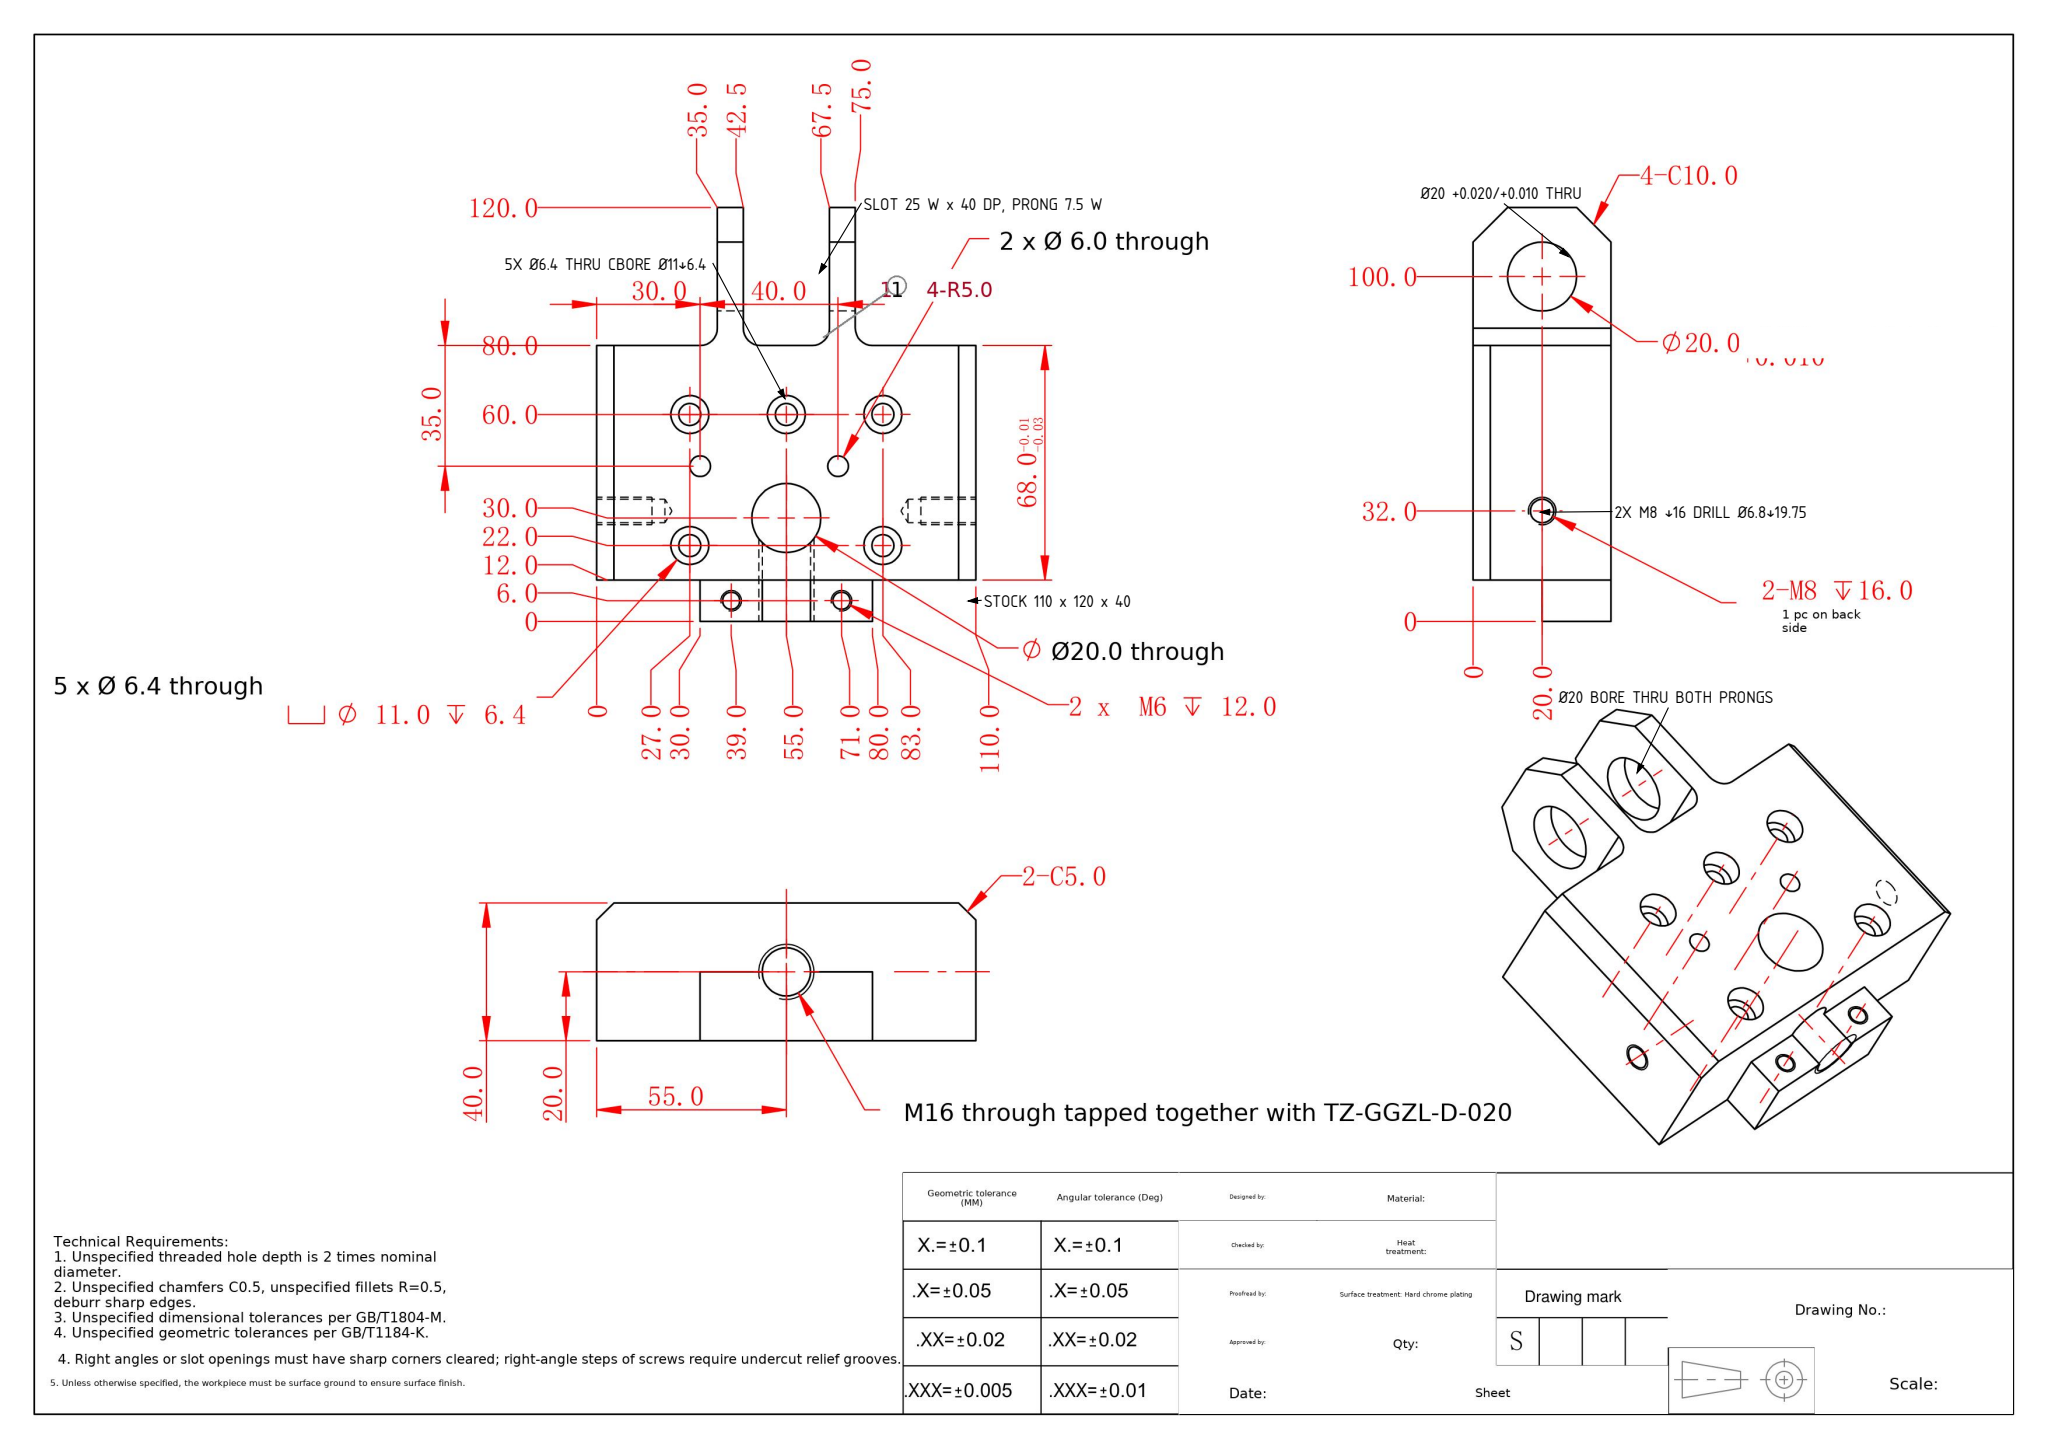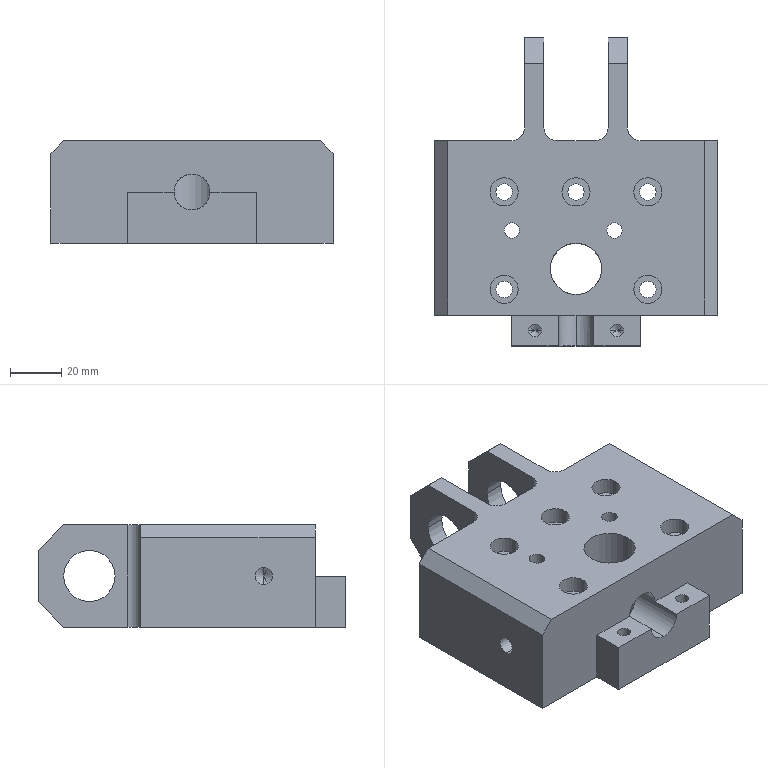Part | SolidWorks | mm | 1 solid | 82 faces | box 110 x 120 x 40 mm | volume 300523 mm3 | cylinder 44 | plane 30 | cone 8 | commonest cylinder face diameters 11 x10 6.4 x10 20 x6 6 x4 6.8 x4 5 x4 10 x4 14 x2
Drawing notes:
STOCK ENVELOPE 110 x 120 x 40 | from the solid: bbox_xyz 110.0,120.0,40.0
TOP PRONGS 7.5 WIDE x 40 HIGH FROM Y80; SLOT BETWEEN 25 WIDE x 40 DEEP | from the solid: x planes 35/42.5 and 67.5/75 = 7.5 wide prongs, 25 gap; y planes 80 to 120 = 40
2-M8 DP 16 TAP DRILL Ø6.8 DP 19.75, 118° PT; CL Y32, Z20, 1 PC EACH SIDE | from the solid: cylinders Ø6.8 axis x at y=32 z=20 len 19.75 (x4) with cones 118° ref dia 6.8
Ø20.0 +0.020/+0.010 BORE THRU BOTH TOP PRONGS, AXIS PARALLEL TO X AT Y=100.0, Z=20.0 FROM MIN-CORNER DATUM | from the solid: cylinders: [20.0,"x",[null,100.0,20.0],7.5, count 4] — coaxial bore through the two 7.5 wide prongs
Ø20.0 (+0.020/+0.010) THRU both top prongs, axis parallel to X at Y=100.0, Z=20.0 from part min corner | from the solid: cylinders[20.0,'x',[null,100.0,20.0],7.5,4]
5X Ø6.4 THRU, C'BORE Ø11.0 DP 6.4 from top face (Z=40); centers at (27,22), (27,60), (55,60), (83,22), (83,60) from min corner | from the solid: cylinders[6.4,'z',...,33.6] and [11.0,'z',...,6.4]
build123d program:
from build123d import *

# Parameters (mm, degrees)
SKETCH1_W                                       = 110
SKETCH1_H                                       = 120
BOSS_EXTRUDE1_DEPTH                             = 20
SKETCH2_W                                       = 35
SKETCH2_H                                       = 40
SKETCH2_W_2                                     = 25
CUT_EXTRUDE1_DEPTH                              = 91.692
SKETCH3_R                                       = 10
CUT_EXTRUDE2_DEPTH                              = 99.107
CHAMFER1_SIZE                                   = 10
FILLET1_R                                       = 5
SKETCH7_R                                       = 10
CUT_EXTRUDE4_DEPTH                              = 91.692
M16_TAPPED_HOLE1_REACH                          = 135.51
M16_TAPPED_HOLE1_BORE_R                         = 7
SKETCH13_W                                      = 110
SKETCH13_H                                      = 12
CUT_EXTRUDE5_DEPTH                              = 20
M6_TAPPED_HOLE1_D                               = 5
M6_TAPPED_HOLE1_DEPTH                           = 15
M6_TAPPED_HOLE1_TIP                             = 1.502
SKETCH16_W                                      = 30
SKETCH16_H                                      = 12
CUT_EXTRUDE6_DEPTH                              = 84.815
CHAMFER2_SIZE                                   = 5
M6_HEX_SOCKET_HEAD_CAP_SCREW_CBORE1_D           = 6.4
M6_HEX_SOCKET_HEAD_CAP_SCREW_CBORE1_CBORE_D     = 11
M6_HEX_SOCKET_HEAD_CAP_SCREW_CBORE1_CBORE_DEPTH = 6.4
F_6_0_6_DIAMETER_HOLE1_D                        = 6


with BuildPart() as part:
    # Sketch1 → Boss-Extrude1 (new, symmetric)
    with BuildSketch(Plane.XY):
        Rectangle(SKETCH1_W, SKETCH1_H)
    extrude(amount=BOSS_EXTRUDE1_DEPTH, both=True)

    # Sketch2 → Cut-Extrude1 (cut, through all)
    with BuildSketch(Plane.XY.offset(20)):
        with Locations((-37.5, 40)):
            Rectangle(SKETCH2_W, SKETCH2_H)
        with Locations((37.5, 40)):
            Rectangle(SKETCH2_W, SKETCH2_H)
        with Locations((0, 40)):
            Rectangle(SKETCH2_W_2, SKETCH2_H)
    extrude(amount=-CUT_EXTRUDE1_DEPTH, mode=Mode.SUBTRACT)

    # Sketch3 → Cut-Extrude2 (cut, through all)
    with BuildSketch(Plane(origin=(20, 0, 0), x_dir=(0, 0, -1), z_dir=(1, 0, 0))):
        with Locations(Location((0, 40, 0), (0, 0, 90))):
            Circle(SKETCH3_R)
    extrude(amount=-CUT_EXTRUDE2_DEPTH, mode=Mode.SUBTRACT)

    # Chamfer1
    chamfer1_edges = [part.edges().sort_by_distance(p)[0] for p in [
        (16.25, 60, -20),
        (16.25, 60, 20),
        (-16.25, 60, -20),
        (-16.25, 60, 20),
    ]]
    chamfer(chamfer1_edges, length=CHAMFER1_SIZE)

    # Fillet1
    fillet1_edges = [part.edges().sort_by_distance(p)[0] for p in [
        (-20, 20, 0),
        (20, 20, 0),
        (-12.5, 20, 0),
        (12.5, 20, 0),
    ]]
    fillet(fillet1_edges, radius=FILLET1_R)

    # Sketch7 → Cut-Extrude4 (cut, through all)
    with BuildSketch(Plane.XY.offset(20)):
        with Locations((0, -30)):
            Circle(SKETCH7_R)
    extrude(amount=-CUT_EXTRUDE4_DEPTH, mode=Mode.SUBTRACT)

    # M16 Tapped Hole1 bore → M16 Tapped Hole1 (cut, up to next)
    with BuildSketch(Plane(origin=(0, -60, 0), x_dir=(-1, 0, 0), z_dir=(0, -1, 0)), mode=Mode.PRIVATE) as m16_tapped_hole1_sk1:
        Circle(M16_TAPPED_HOLE1_BORE_R)
    m16_tapped_hole1_tool1 = extrude(m16_tapped_hole1_sk1.sketch, amount=-M16_TAPPED_HOLE1_REACH, mode=Mode.PRIVATE) & part.part
    add(m16_tapped_hole1_tool1.solids().sort_by_distance((0, -60, 0))[0], mode=Mode.SUBTRACT)

    # Sketch13 → Cut-Extrude5 (cut)
    with BuildSketch(Plane.XY.offset(20)):
        with Locations((0, -54)):
            Rectangle(SKETCH13_W, SKETCH13_H)
    extrude(amount=-CUT_EXTRUDE5_DEPTH, mode=Mode.SUBTRACT)

    # M6 Tapped Hole1
    with Locations(Plane.XY):
        with Locations((-16, -54), (16, -54)):
            Hole(M6_TAPPED_HOLE1_D / 2, depth=M6_TAPPED_HOLE1_DEPTH)
            with Locations((0, 0, -(M6_TAPPED_HOLE1_DEPTH + M6_TAPPED_HOLE1_TIP / 2))):  # 118° drill point
                Cone(0, M6_TAPPED_HOLE1_D / 2, M6_TAPPED_HOLE1_TIP, mode=Mode.SUBTRACT)

    # Sketch16 → Cut-Extrude6 (cut, through all)
    with BuildSketch(Plane.XY):
        with Locations((-40, -54)):
            Rectangle(SKETCH16_W, SKETCH16_H)
        with Locations((40, -54)):
            Rectangle(SKETCH16_W, SKETCH16_H)
    extrude(amount=-CUT_EXTRUDE6_DEPTH, mode=Mode.SUBTRACT)

    # Sketch17 → M8 Tapped Hole1 (revolve, cut)
    with BuildSketch(Plane(origin=(-55, -28, 0), x_dir=(0, 0, 1), z_dir=(0, 1, 0))):
        Polygon((0, 0), (0, 21.793), (3.4, 19.75), (3.4, 0), align=None)
    m8_tapped_hole1 = revolve(axis=Axis((-61.35, -28, 0), (1, 0, 0)), mode=Mode.SUBTRACT)

    # Mirror1: M8 Tapped Hole1 across plane
    add(m8_tapped_hole1.mirror(Plane(origin=(0, 0, 0), x_dir=(0, 0, 1), z_dir=(1, 0, 0))), mode=Mode.SUBTRACT)

    # Chamfer2
    chamfer2_edges = [part.edges().sort_by_distance(p)[0] for p in [
        (55, -14, 20),
        (-55, -14, 20),
    ]]
    chamfer(chamfer2_edges, length=CHAMFER2_SIZE)

    # M6 Hex Socket Head Cap Screw CBORE1 (through all)
    with Locations(Plane.XY.offset(20)):
        with Locations((-28, -38), (-28, 0), (0, 0), (28, 0), (28, -38)):
            CounterBoreHole(M6_HEX_SOCKET_HEAD_CAP_SCREW_CBORE1_D / 2, M6_HEX_SOCKET_HEAD_CAP_SCREW_CBORE1_CBORE_D / 2, M6_HEX_SOCKET_HEAD_CAP_SCREW_CBORE1_CBORE_DEPTH)

    # 6.0 _6_ Diameter Hole1 (through all)
    with Locations(Plane.XY.offset(20)):
        with Locations((-25, -15), (15, -15)):
            Hole(F_6_0_6_DIAMETER_HOLE1_D / 2)


solid = part.part